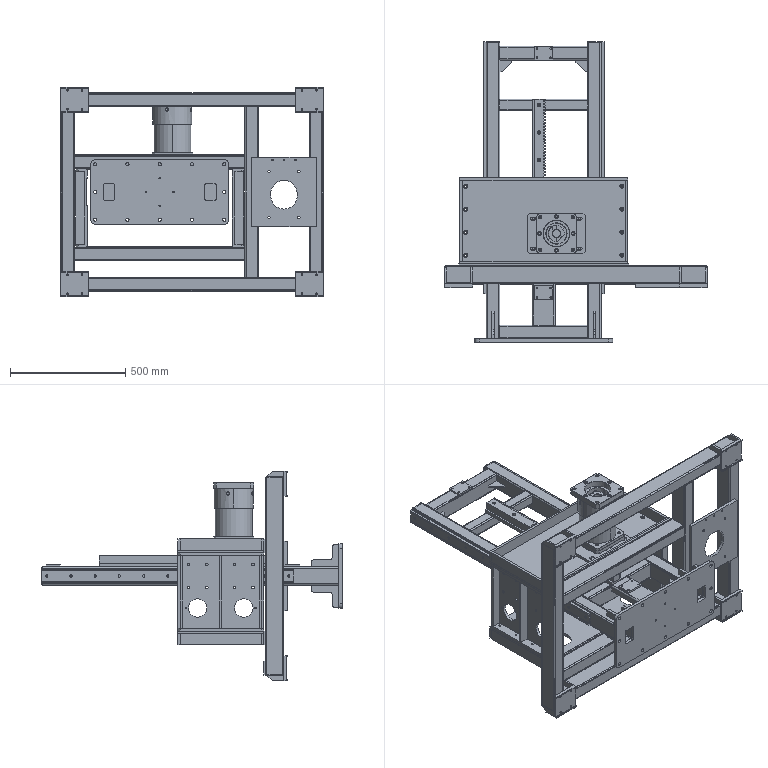Assembly | SolidWorks | mm | 15 component files | 77 solids | 2532 faces | box 1138 x 1305 x 910 mm | volume 34633737 mm3 | plane 1142 | cylinder 935 | torus 178 | cone 104 | sphere 104 | spline 69 | commonest cylinder face diameters 10.2 x138 6.8 x108 8.5 x80 12 x69 11 x60 18 x52 14 x50 6 x48
Bill of materials:
BearingRetainingRing | 1 |  | Thin flat plain annular ring (washer- or shim-like) with a rectangular cross-section.
Rolling bearings 6012 GB 276-94 | 2 |  | Thin-section annular ball-bearing-like geometry: a concentric outer ring and inner ring with a single row of spherical balls between them. Both faces are open (no shields or seals), and the bore is a plain cylinder.
DriveGearPart | 1 |  | Spur gear with an integral cylindrical hub on one side. It has a keyed through-bore and a small circumferential groove near the top of the hub.
DriveRackPart | 1 |  | Long straight rectangular bar with straight teeth along one long edge (gear-rack-like). A row of evenly spaced through holes runs along the flat face.
MovingVerticalPlate1 | 2 |  | Thick rectangular plate or block with two large round through holes in its lower half and a grid of small holes. It has a stepped or recessed profile across the faces and a chamfered edge.
MovingVerticalPlate2 | 1 |  | Rectangular flat plate with two round through holes, two rectangular through cutouts with rounded corners, and small holes along both short ends. Edge holes are also drilled into the side faces.
MovingVerticalPlate3 | 1 |  | Shallow rectangular tray or pocketed plate: a raised perimeter wall around a flat floor. It has one large central round through hole surrounded by four small holes, plus small holes along the ends and side walls.
PlanetaryReducer-PLF142 | 1 |  | Cylindrical housing with square flanges at both ends and a projecting output shaft at one end. It looks like a gearhead or reducer-type unit.
PlanetaryReducer-PLF142BearingHousing | 1 |  | Square flange with chamfered corners, four through holes and a central bore. A stepped cylindrical spigot or boss projects from one face.
PlanetaryReducer-PLF142Mount1 | 1 |  | Flat rectangular plate with chamfered corners, a large central round through hole and four elongated slots, one near each corner.
shaft circlip GB894-1 d60 | 1 |  | Thin flat split ring with two lugs at the gap, each with a small hole. This shape resembles an external retaining ring.
SupportFrame1 | 1 |  | Rectangular planar frame of beam members with corner mounting pads. It has two horizontal cross-members on one side and a vertical member carrying a plate with a large round hole and a small-hole pattern.
UprightFrame | 1 |  | Long rectangular ladder-type frame with several cross-members, attached at one end to a large plate. A longitudinal slotted strip or rail runs along the center and one side member.
Mates:
1. coincident | SupportFrame1-1 face at (0, 48, 0) dir (0, 1, 0) | MovingVerticalPlate2-1 face at (224, 48, -299) dir (0, -1, 0)
2. concentric | SupportFrame1-1 face at (180, 48, -269) dir (0, 1, 0) r 4.25 | MovingVerticalPlate2-1 face at (180, 58, -269) dir (0, 1, 0) r 5.5
3. parallel | SupportFrame1-1 face at (259, 34, -299) dir (0, 0, -1) | MovingVerticalPlate2-1 face at (-140, 234, -299) dir (0, 0, -1)
4. coincident | MovingVerticalPlate2-1 face at (-504, 48, -239) dir (0, 0, 1) | MovingVerticalPlate1-1 face at (-504, 48, -239) dir (0, 0, -1)
5. coincident | MovingVerticalPlate2-1 face at (-457, 48, -236) dir (-1, 0, 0) | MovingVerticalPlate1-1 face at (-457, 48, -239) dir (1, 0, 0)
6. concentric | MovingVerticalPlate2-1 face at (-479, 384, -248) dir (0, 0, -1) r 5.5 | MovingVerticalPlate1-1 face at (-479, 384, -239) dir (0, 0, -1) r 4.25
7. concentric | MovingVerticalPlate2-1 face at (199, 384, -248) dir (0, 0, -1) r 5.5 | MovingVerticalPlate1-2 face at (199, 384, -239) dir (0, 0, -1) r 4.25
8. parallel | MovingVerticalPlate2-1 face at (224, 420, -248) dir (1, 0, 0) | MovingVerticalPlate1-2 face at (174, 420, -239) dir (-1, 0, 0)
9. coincident | MovingVerticalPlate2-1 face at (224, 48, -239) dir (0, 0, 1) | MovingVerticalPlate1-2 face at (224, 420, -239) dir (0, 0, -1)
10. parallel | SupportFrame1-1 face at (539, -34, 430) dir (0, 0, 1) | UprightFrame-1 face at (80, 985.363, 40) dir (0, 0, 1)
11. width | MovingVerticalPlate1-1 face at (-454, 48, -239) dir (1, 0, 0) | MovingVerticalPlate1-2 face at (174, 420, -239) dir (-1, 0, 0) | UprightFrame-1 face at (-330, 1011.363, -34) dir (1, 0, 0) | UprightFrame-1 face at (50, 1011.363, 34) dir (-1, 0, 0)
12. coincident | UprightFrame-1 face at (-140, -278.637, 50.5) dir (0, 0, 1) | DriveRackPart-1 face at (-180, -13.637, 50.5) dir (0, 0, -1)
13. coincident | UprightFrame-1 face at (-180, 761.363, 55) dir (1, 0, 0) | DriveRackPart-1 face at (-180, -13.637, 50.5) dir (-1, 0, 0)
14. concentric | UprightFrame-1 face at (-160, 736.363, 50.5) dir (0, 0, 1) r 3.4 | DriveRackPart-1 face at (-160, 736.363, 88.5) dir (0, 0, 1) r 7.5
15. coincident | SupportFrame1-1 face at (0, 48, 0) dir (0, 1, 0) | MovingVerticalPlate3-1 face at (-504, 48, 161) dir (0, -1, 0)
16. concentric | SupportFrame1-1 face at (-460, 48, 131) dir (0, 1, 0) r 4.25 | MovingVerticalPlate3-1 face at (-460, 58, 131) dir (0, 1, 0) r 5.5
17. concentric | SupportFrame1-1 face at (180, 48, 131) dir (0, 1, 0) r 4.25 | MovingVerticalPlate3-1 face at (180, 58, 131) dir (0, 1, 0) r 5.5
18. distance | PlanetaryReducer-PLF142-1 face at (-10.376, 265.5, 171) dir (0, 1, 0) | SupportFrame1-1 face at (-515, 40, 400) dir (0, 1, 0)
19. distance | PlanetaryReducer-PLF142-1 face at (-172.5, 103.376, 171) dir (-1, 0, 0) | SupportFrame1-1 face at (-569, -34, 400) dir (-1, 0, 0)
20. distance | PlanetaryReducer-PLF142-1 face at (1.5, 91.5, 172) dir (0, 0, 1) | MovingVerticalPlate3-1 face at (-140, 234, 161) dir (0, 0, 1)
21. concentric | PlanetaryReducer-PLF142-1 face at (-85, 178, 71) dir (0, 0, 1) r 20 | DriveGearPart-1 face at (-85, 178, 146) dir (0, 0, -1) r 30
22. width | DriveRackPart-1 face at (-180, -13.637, 88.5) dir (0, 0, 1) | DriveRackPart-1 face at (-180, -13.637, 50.5) dir (0, 0, -1) | DriveGearPart-1 face at (-85, 178, 87) dir (0, 0, 1) | DriveGearPart-1 face at (-85, 178, 52) dir (0, 0, -1)
23. rack pinion | DriveRackPart-1 sketch segment at (-144.754, -13.637, 88.5) dir (0, 1, 0) | DriveGearPart-1 sketch segment at (-85, 178, 87) dir (0, 0, 1) r 52.5
24. concentric | DriveGearPart-1 face at (-85, 178, 146) dir (0, 0, -1) r 30 | PlanetaryReducer-PLF142BearingHousing-1 face at (-85, 178, 122) dir (0, 0, -1) r 57.5
25. concentric | PlanetaryReducer-PLF142BearingHousing-1 face at (-85, 178, 122) dir (0, 0, -1) r 57.5 | PlanetaryReducer-PLF142Mount1-1 face at (-85, 178, 110) dir (0, 0, 1) r 57.75
26. coincident | PlanetaryReducer-PLF142BearingHousing-1 face at (-85, 178, 122) dir (0, 0, -1) | PlanetaryReducer-PLF142Mount1-1 face at (-85, 178, 122) dir (0, 0, 1)
27. coincident | PlanetaryReducer-PLF142-1 face at (1.5, 91.5, 157) dir (0, 0, -1) | PlanetaryReducer-PLF142BearingHousing-1 face at (-85, 178, 157) dir (0, 0, 1)
28. coincident | PlanetaryReducer-PLF142-1 face at (-172.5, 103.376, 171) dir (-1, 0, 0) | PlanetaryReducer-PLF142BearingHousing-1 face at (-172.5, 90.5, 157) dir (-1, 0, 0)
29. parallel | PlanetaryReducer-PLF142-1 face at (-10.376, 265.5, 171) dir (0, 1, 0) | PlanetaryReducer-PLF142Mount1-1 face at (-210, 265.5, 122) dir (0, 1, 0)
30. concentric | DriveGearPart-1 face at (-85, 178, 146) dir (0, 0, -1) r 30 | deep groove ball bearings gb-1 face at (-85, 178, 112.971) dir (0, 0, 1) r 30
31. coincident | PlanetaryReducer-PLF142BearingHousing-1 face at (-85, 178, 97) dir (0, 0, 1) | deep groove ball bearings gb-1 face at (-113.492, 216.006, 97) dir (0, 0, -1)
32. concentric | deep groove ball bearings gb-1 face at (-85, 178, 112.971) dir (0, 0, 1) r 30 | deep groove ball bearings gb-2 face at (-85, 178, 134.971) dir (0, 0, 1) r 30
33. concentric | deep groove ball bearings gb-2 face at (-85, 178, 136.711) dir (0, 0, 1) r 47.5 | BearingRetainingRing-1 face at (-85, 178, 115) dir (0, 0, 1) r 35
34. coincident | deep groove ball bearings gb-1 face at (-106.494, 206.671, 115) dir (0, 0, 1) | BearingRetainingRing-1 face at (-85, 178, 115) dir (0, 0, -1)
35. coincident | deep groove ball bearings gb-2 face at (-93.779, 206.687, 119) dir (0, 0, -1) | BearingRetainingRing-1 face at (-85, 178, 119) dir (0, 0, 1)
36. distance | MovingVerticalPlate1-1 face at (-454, 420, -69) dir (0, 1, 0) | UprightFrame-1 face at (-335.5, 1011.363, -34.5) dir (0, 1, 0)
37. concentric | DriveGearPart-1 face at (-85, 178, 52) dir (0, 0, -1) r 28.5 | shaft circlip GB894-1 d60-1 face at (-85, 178, 141) dir (0, 0, -1) r 28.5
38. coincident | DriveGearPart-1 face at (-85, 208, 139) dir (0, 0, 1) | shaft circlip GB894-1 d60-1 face at (-85, 178, 139) dir (0, 0, -1)